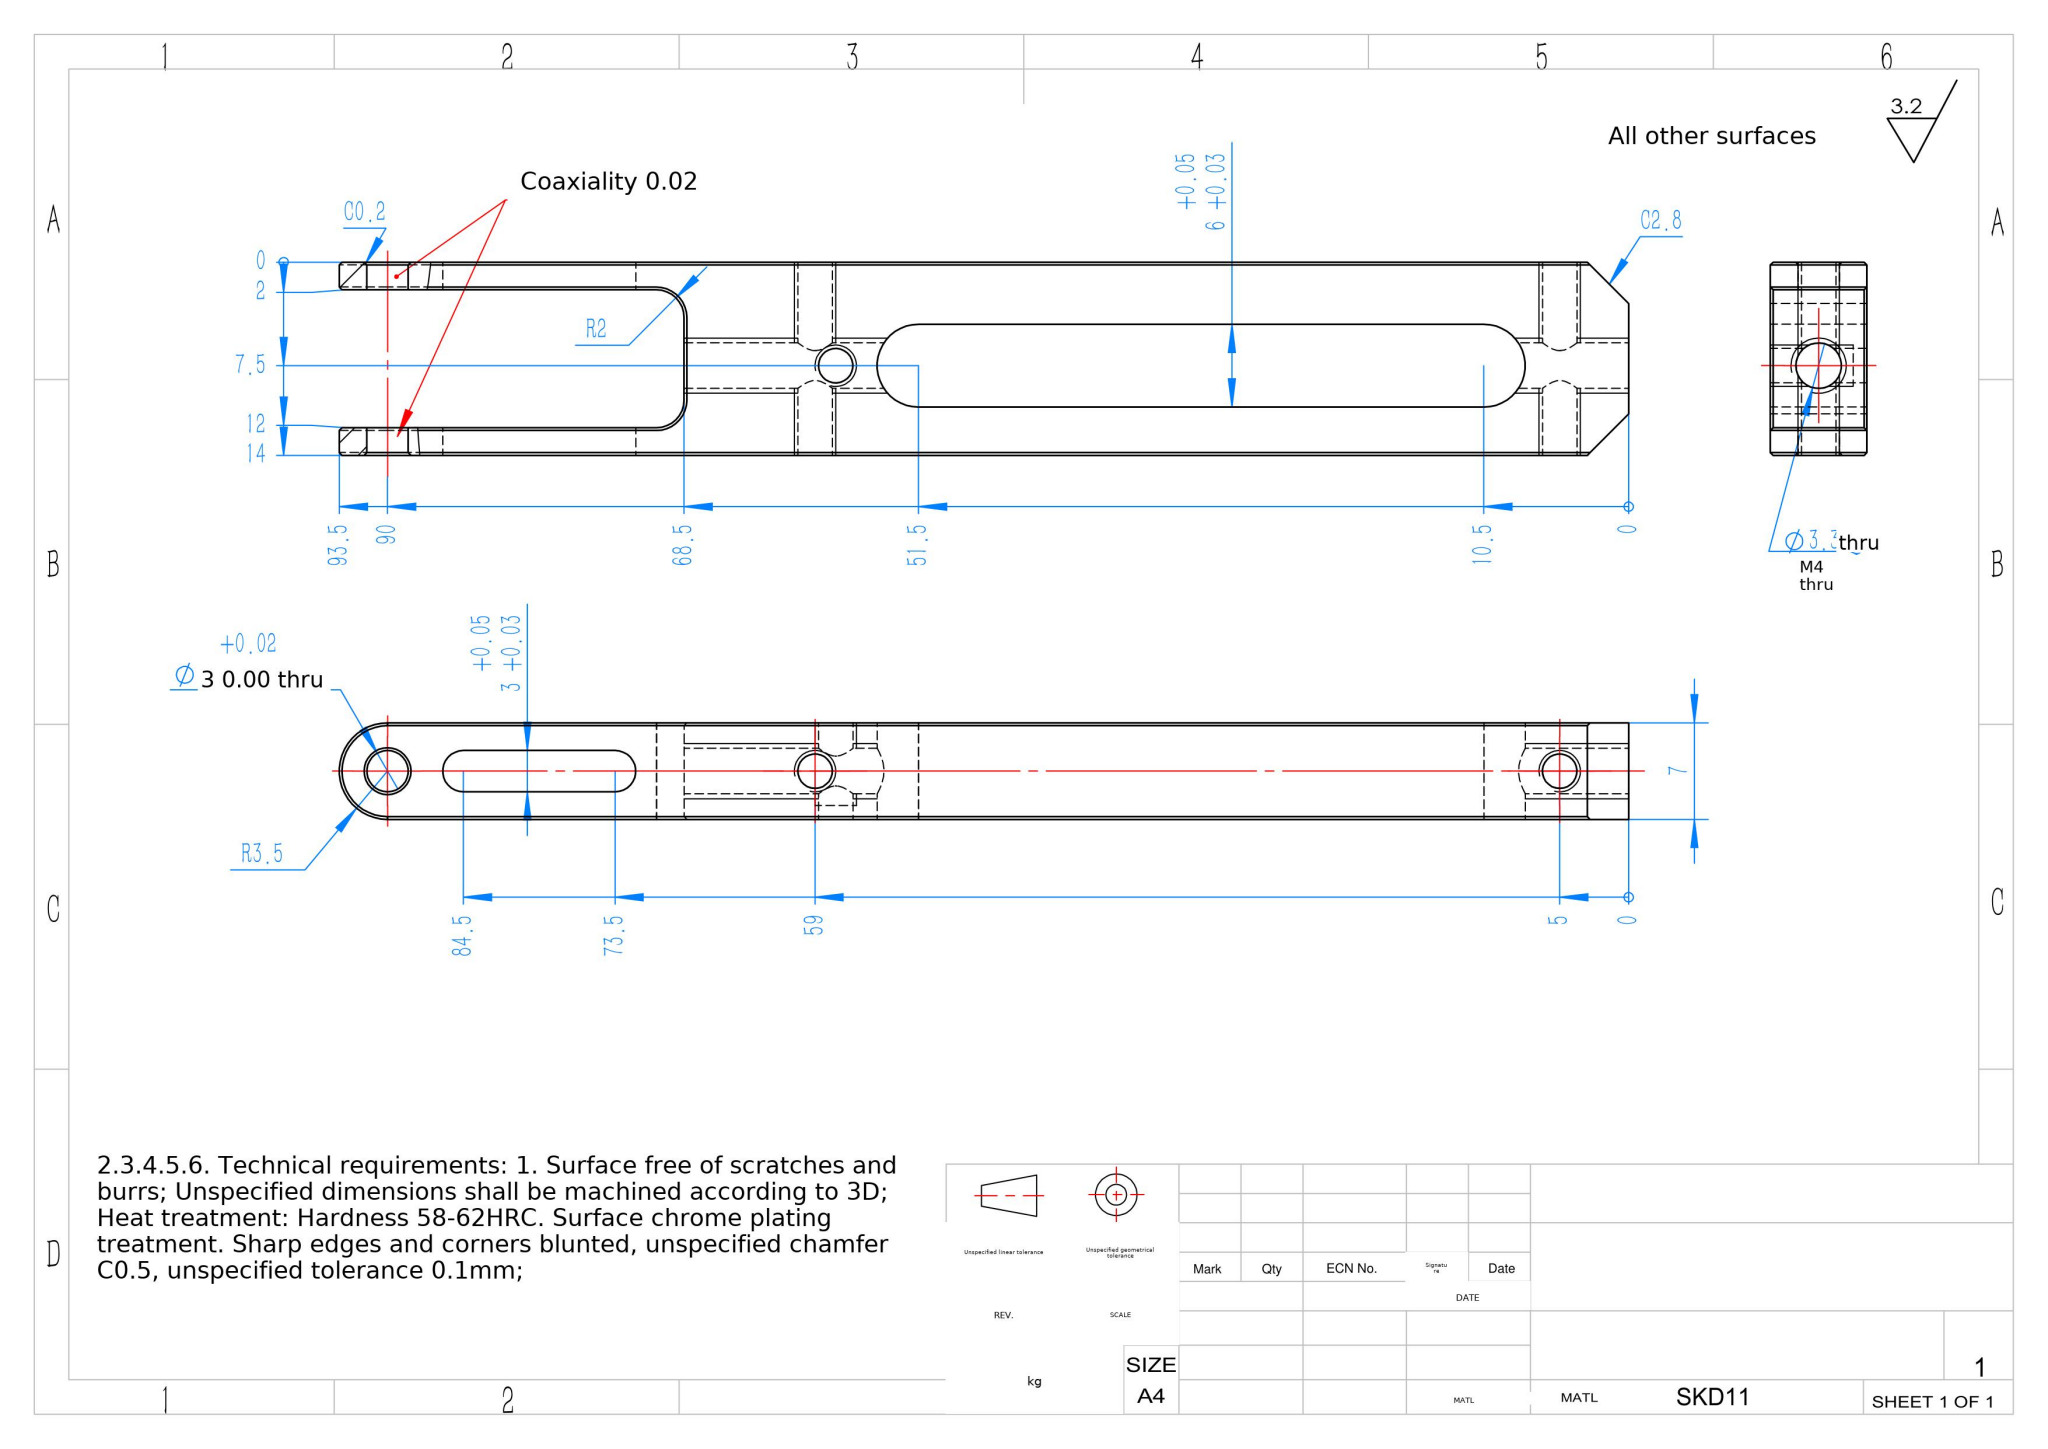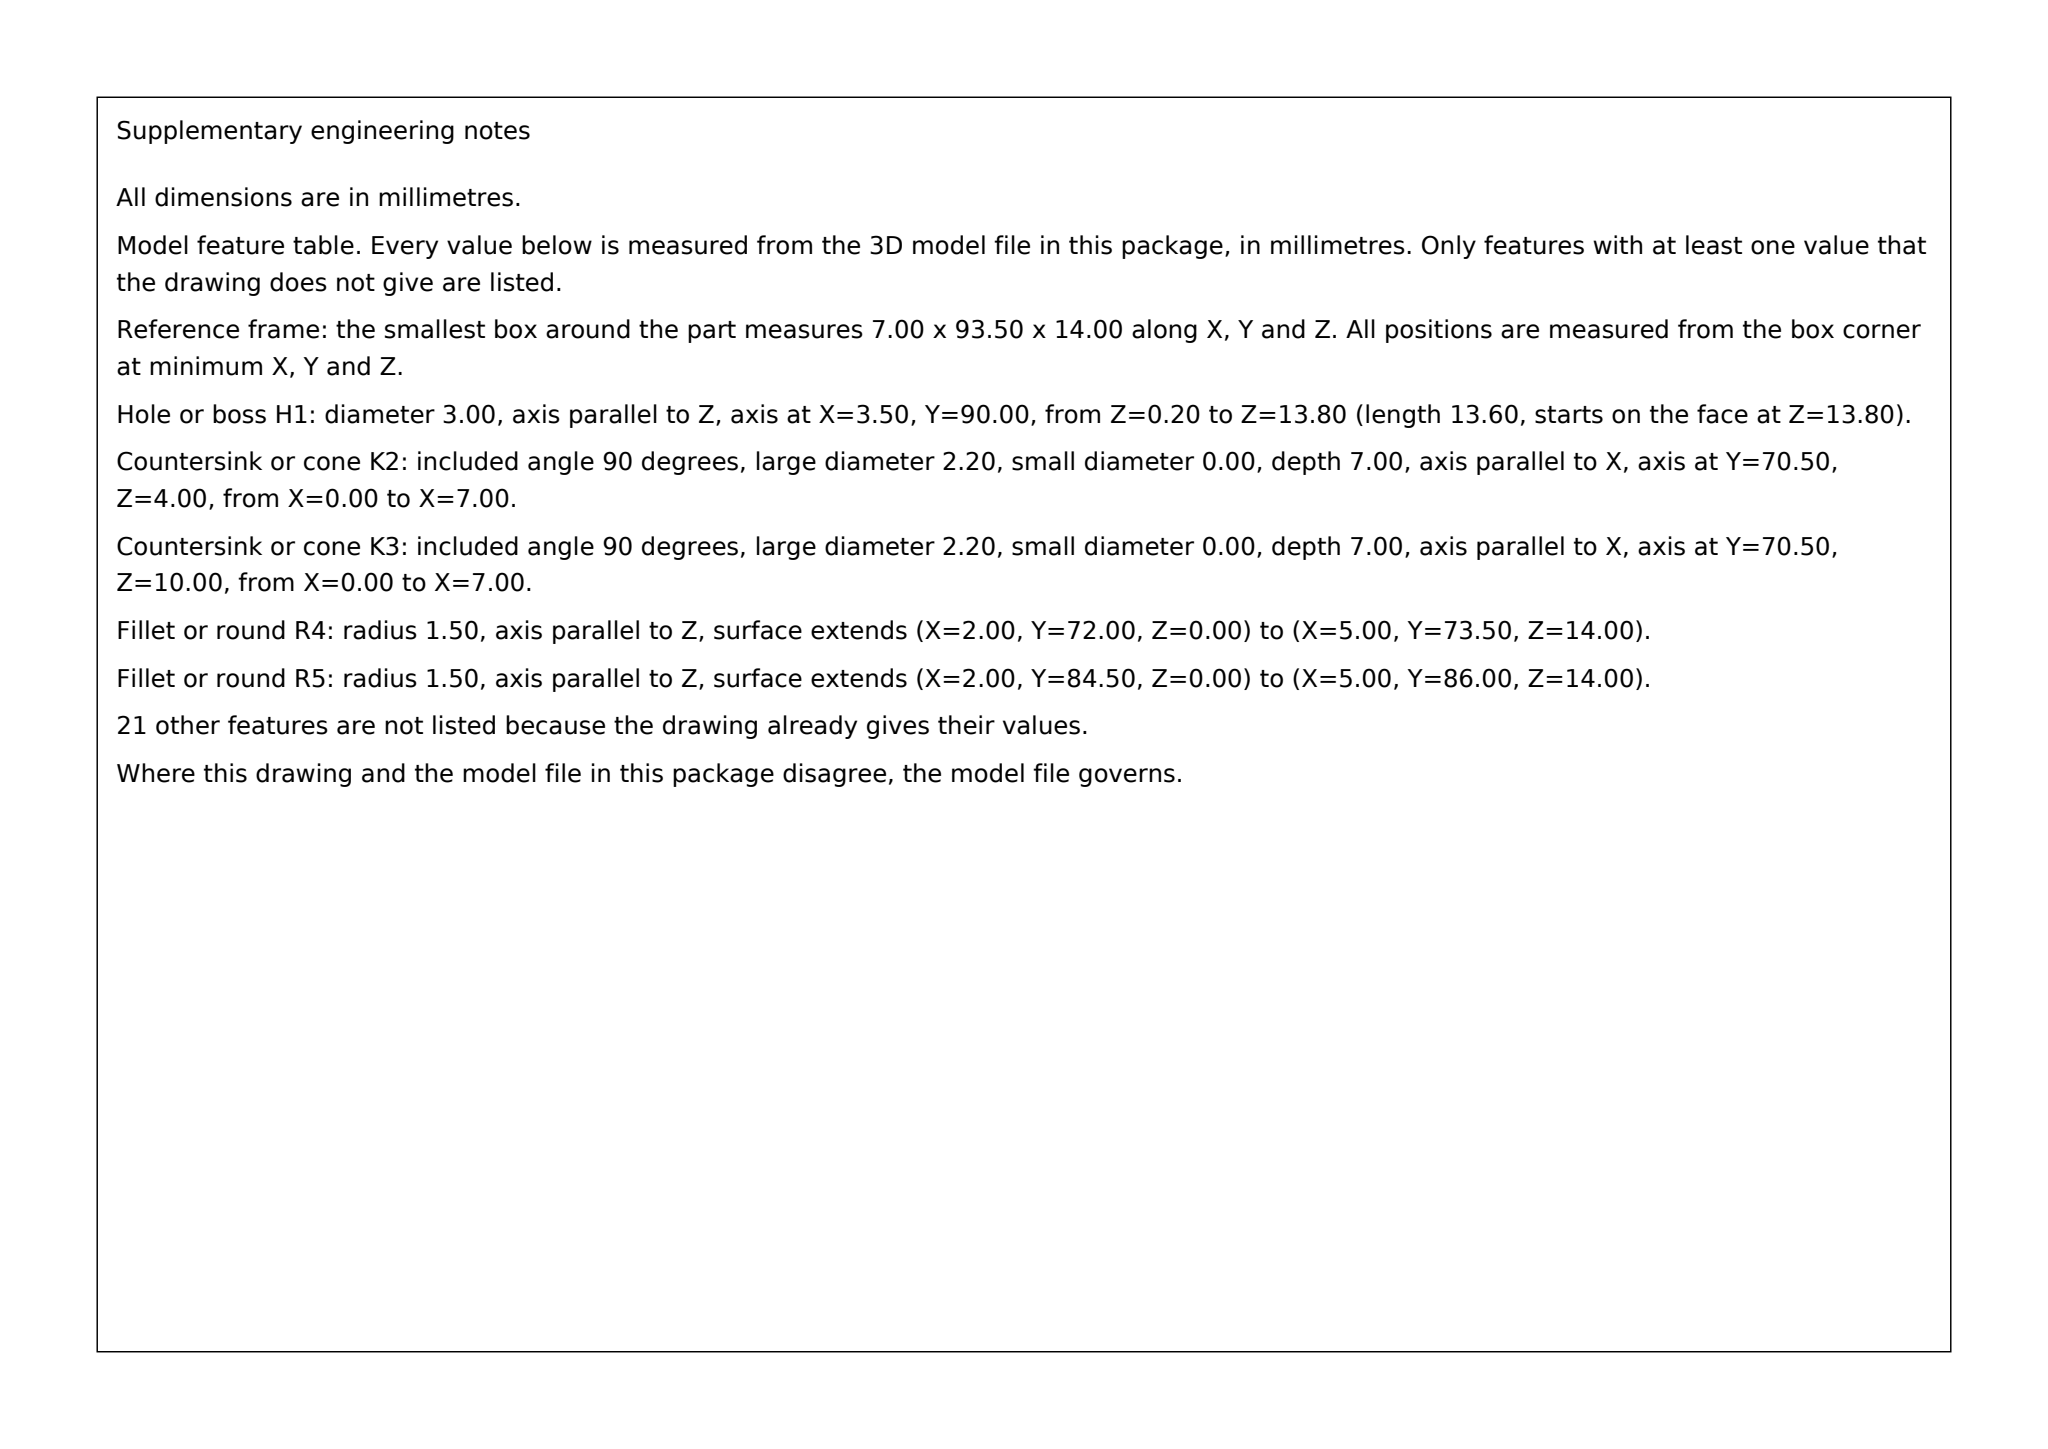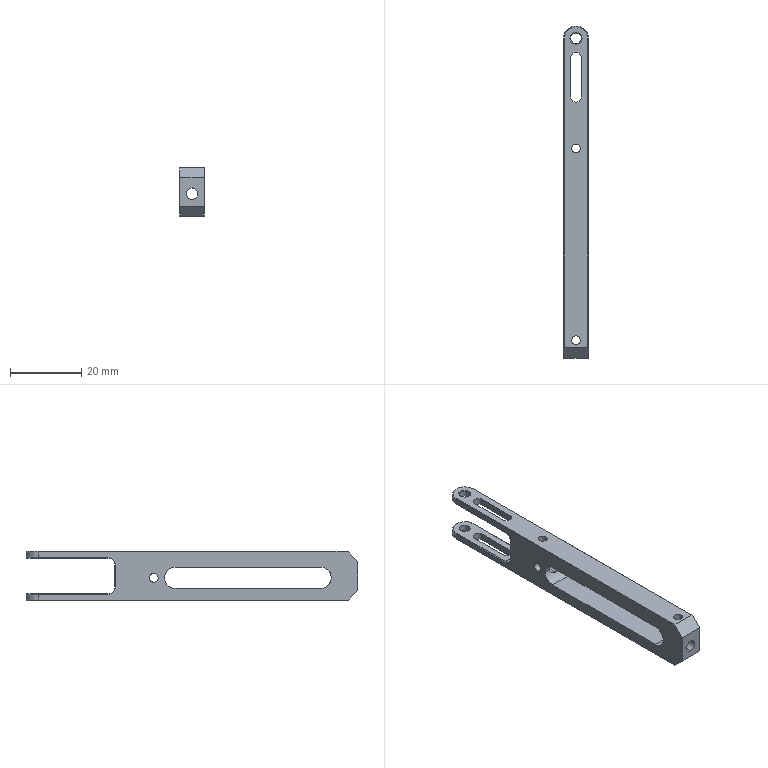Part | SolidWorks | mm | material SKD11 | 1 solid | 69 faces | box 7 x 93.5 x 14 mm | volume 4909 mm3 | cylinder 31 | plane 26 | cone 12 | commonest cylinder face diameters 2.5 x12 3 x8 3.3 x4 6 x3 7 x2 4 x2